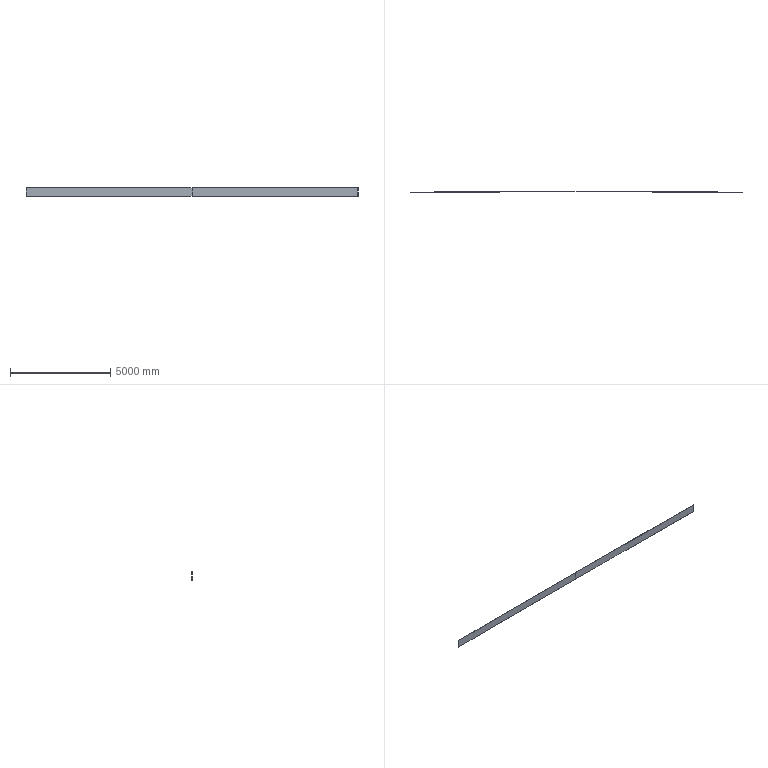Component | SolidWorks | UpperCover-1 | 1 solid | 8 faces | box 16590 x 30 x 400 mm | volume 66360064 mm3 | cylinder 4 | plane 4 | commonest cylinder face diameters 3440371.25 x2 3440351.25 x2 | material Plain Carbon Steel
STEP:
#1=COLOUR_RGB('',0.7922,0.8196,0.9333);
#2=FILL_AREA_STYLE_COLOUR('',#1);
#3=FILL_AREA_STYLE('',(#2));
#4=SURFACE_STYLE_FILL_AREA(#3);
#5=SURFACE_SIDE_STYLE('',(#4));
#6=SURFACE_STYLE_USAGE(.BOTH.,#5);
#7=PRESENTATION_STYLE_ASSIGNMENT((#6));
#8=CARTESIAN_POINT('',(18.305,126.764,80.917));
#9=VERTEX_POINT('',#8);
#10=CARTESIAN_POINT('',(344.879,127.551,80.917));
#11=VERTEX_POINT('',#10);
#12=CARTESIAN_POINT('',(344.879,-67596.292,80.917));
#13=DIRECTION('',(-0.,0.,-1.));
#14=DIRECTION('',(-0.,1.,0.));
#15=AXIS2_PLACEMENT_3D('',#12,#13,#14);
#16=CIRCLE('',#15,67723.844);
#17=EDGE_CURVE('',#9,#11,#16,.T.);
#18=ORIENTED_EDGE('',*,*,#17,.T.);
#19=CARTESIAN_POINT('',(344.879,127.551,65.169));
#20=VERTEX_POINT('',#19);
#21=CARTESIAN_POINT('',(344.879,127.551,80.917));
#22=DIRECTION('',(-0.,0.,-1.));
#23=VECTOR('',#22,39.37);
#24=LINE('',#21,#23);
#25=EDGE_CURVE('',#11,#20,#24,.T.);
#26=ORIENTED_EDGE('',*,*,#25,.T.);
#27=CARTESIAN_POINT('',(18.305,126.764,65.169));
#28=VERTEX_POINT('',#27);
#29=CARTESIAN_POINT('',(344.879,-67596.292,65.169));
#30=DIRECTION('',(-0.,0.,-1.));
#31=DIRECTION('',(-0.,1.,0.));
#32=AXIS2_PLACEMENT_3D('',#29,#30,#31);
#33=CIRCLE('',#32,67723.844);
#34=EDGE_CURVE('',#28,#20,#33,.T.);
#35=ORIENTED_EDGE('',*,*,#34,.F.);
#36=CARTESIAN_POINT('',(18.305,126.764,80.917));
#37=DIRECTION('',(-0.,0.,-1.));
#38=VECTOR('',#37,39.37);
#39=LINE('',#36,#38);
#40=EDGE_CURVE('',#9,#28,#39,.T.);
#41=ORIENTED_EDGE('',*,*,#40,.F.);
#42=EDGE_LOOP('',(#18,#26,#35,#41));
#43=FACE_OUTER_BOUND('',#42,.T.);
#44=CARTESIAN_POINT('',(344.879,-67596.292,80.917));
#45=DIRECTION('',(-0.,0.,-1.));
#46=DIRECTION('',(-0.,1.,0.));
#47=AXIS2_PLACEMENT_3D('',#44,#45,#46);
#48=CYLINDRICAL_SURFACE('',#47,67723.844);
#49=ADVANCED_FACE('',(#43),#48,.T.);
#50=CARTESIAN_POINT('',(344.879,127.158,80.917));
#51=VERTEX_POINT('',#50);
#52=CARTESIAN_POINT('',(671.452,126.37,80.917));
#53=VERTEX_POINT('',#52);
#54=CARTESIAN_POINT('',(344.879,-67596.292,80.917));
#55=DIRECTION('',(-0.,0.,-1.));
#56=DIRECTION('',(1.,0.,-0.));
#57=AXIS2_PLACEMENT_3D('',#54,#55,#56);
#58=CIRCLE('',#57,67723.45);
#59=EDGE_CURVE('',#51,#53,#58,.T.);
#60=ORIENTED_EDGE('',*,*,#59,.F.);
#61=CARTESIAN_POINT('',(344.879,127.158,65.169));
#62=VERTEX_POINT('',#61);
#63=CARTESIAN_POINT('',(344.879,127.158,80.917));
#64=DIRECTION('',(-0.,0.,-1.));
#65=VECTOR('',#64,39.37);
#66=LINE('',#63,#65);
#67=EDGE_CURVE('',#51,#62,#66,.T.);
#68=ORIENTED_EDGE('',*,*,#67,.T.);
#69=CARTESIAN_POINT('',(671.452,126.37,65.169));
#70=VERTEX_POINT('',#69);
#71=CARTESIAN_POINT('',(344.879,-67596.292,65.169));
#72=DIRECTION('',(-0.,0.,-1.));
#73=DIRECTION('',(1.,0.,-0.));
#74=AXIS2_PLACEMENT_3D('',#71,#72,#73);
#75=CIRCLE('',#74,67723.45);
#76=EDGE_CURVE('',#62,#70,#75,.T.);
#77=ORIENTED_EDGE('',*,*,#76,.T.);
#78=CARTESIAN_POINT('',(671.452,126.37,80.917));
#79=DIRECTION('',(-0.,0.,-1.));
#80=VECTOR('',#79,39.37);
#81=LINE('',#78,#80);
#82=EDGE_CURVE('',#53,#70,#81,.T.);
#83=ORIENTED_EDGE('',*,*,#82,.F.);
#84=EDGE_LOOP('',(#60,#68,#77,#83));
#85=FACE_OUTER_BOUND('',#84,.T.);
#86=CARTESIAN_POINT('',(344.879,-67596.292,80.917));
#87=DIRECTION('',(-0.,0.,-1.));
#88=DIRECTION('',(-0.,1.,0.));
#89=AXIS2_PLACEMENT_3D('',#86,#87,#88);
#90=CYLINDRICAL_SURFACE('',#89,67723.45);
#91=ADVANCED_FACE('',(#85),#90,.F.);
#92=ORIENTED_EDGE('',*,*,#67,.F.);
#93=CARTESIAN_POINT('',(18.307,126.37,80.917));
#94=VERTEX_POINT('',#93);
#95=CARTESIAN_POINT('',(344.879,-67596.292,80.917));
#96=DIRECTION('',(-0.,0.,-1.));
#97=DIRECTION('',(1.,0.,-0.));
#98=AXIS2_PLACEMENT_3D('',#95,#96,#97);
#99=CIRCLE('',#98,67723.45);
#100=EDGE_CURVE('',#94,#51,#99,.T.);
#101=ORIENTED_EDGE('',*,*,#100,.F.);
#102=CARTESIAN_POINT('',(18.307,126.37,65.169));
#103=VERTEX_POINT('',#102);
#104=CARTESIAN_POINT('',(18.307,126.37,80.917));
#105=DIRECTION('',(-0.,0.,-1.));
#106=VECTOR('',#105,39.37);
#107=LINE('',#104,#106);
#108=EDGE_CURVE('',#94,#103,#107,.T.);
#109=ORIENTED_EDGE('',*,*,#108,.T.);
#110=CARTESIAN_POINT('',(344.879,-67596.292,65.169));
#111=DIRECTION('',(-0.,0.,-1.));
#112=DIRECTION('',(1.,0.,-0.));
#113=AXIS2_PLACEMENT_3D('',#110,#111,#112);
#114=CIRCLE('',#113,67723.45);
#115=EDGE_CURVE('',#103,#62,#114,.T.);
#116=ORIENTED_EDGE('',*,*,#115,.T.);
#117=EDGE_LOOP('',(#92,#101,#109,#116));
#118=FACE_OUTER_BOUND('',#117,.T.);
#119=CARTESIAN_POINT('',(344.879,-67596.292,80.917));
#120=DIRECTION('',(-0.,0.,-1.));
#121=DIRECTION('',(-0.,1.,0.));
#122=AXIS2_PLACEMENT_3D('',#119,#120,#121);
#123=CYLINDRICAL_SURFACE('',#122,67723.45);
#124=ADVANCED_FACE('',(#118),#123,.F.);
#125=CARTESIAN_POINT('',(671.454,126.764,65.169));
#126=VERTEX_POINT('',#125);
#127=CARTESIAN_POINT('',(671.454,126.764,65.169));
#128=DIRECTION('',(-0.004822,-1.,-0.));
#129=VECTOR('',#128,39.37);
#130=LINE('',#127,#129);
#131=EDGE_CURVE('',#126,#70,#130,.T.);
#132=ORIENTED_EDGE('',*,*,#131,.F.);
#133=CARTESIAN_POINT('',(671.454,126.764,80.917));
#134=VERTEX_POINT('',#133);
#135=CARTESIAN_POINT('',(671.454,126.764,80.917));
#136=DIRECTION('',(-0.,0.,-1.));
#137=VECTOR('',#136,39.37);
#138=LINE('',#135,#137);
#139=EDGE_CURVE('',#134,#126,#138,.T.);
#140=ORIENTED_EDGE('',*,*,#139,.F.);
#141=CARTESIAN_POINT('',(671.454,126.764,80.917));
#142=DIRECTION('',(-0.004822,-1.,-0.));
#143=VECTOR('',#142,39.37);
#144=LINE('',#141,#143);
#145=EDGE_CURVE('',#134,#53,#144,.T.);
#146=ORIENTED_EDGE('',*,*,#145,.T.);
#147=ORIENTED_EDGE('',*,*,#82,.T.);
#148=EDGE_LOOP('',(#132,#140,#146,#147));
#149=FACE_OUTER_BOUND('',#148,.T.);
#150=CARTESIAN_POINT('',(671.454,126.764,80.917));
#151=DIRECTION('',(1.,-0.004822,-0.));
#152=DIRECTION('',(0.004822,1.,0.));
#153=AXIS2_PLACEMENT_3D('',#150,#151,#152);
#154=PLANE('',#153);
#155=ADVANCED_FACE('',(#149),#154,.T.);
#156=ORIENTED_EDGE('',*,*,#25,.F.);
#157=CARTESIAN_POINT('',(344.879,-67596.292,80.917));
#158=DIRECTION('',(-0.,0.,-1.));
#159=DIRECTION('',(-0.,1.,0.));
#160=AXIS2_PLACEMENT_3D('',#157,#158,#159);
#161=CIRCLE('',#160,67723.844);
#162=EDGE_CURVE('',#11,#134,#161,.T.);
#163=ORIENTED_EDGE('',*,*,#162,.T.);
#164=ORIENTED_EDGE('',*,*,#139,.T.);
#165=CARTESIAN_POINT('',(344.879,-67596.292,65.169));
#166=DIRECTION('',(-0.,0.,-1.));
#167=DIRECTION('',(-0.,1.,0.));
#168=AXIS2_PLACEMENT_3D('',#165,#166,#167);
#169=CIRCLE('',#168,67723.844);
#170=EDGE_CURVE('',#20,#126,#169,.T.);
#171=ORIENTED_EDGE('',*,*,#170,.F.);
#172=EDGE_LOOP('',(#156,#163,#164,#171));
#173=FACE_OUTER_BOUND('',#172,.T.);
#174=CARTESIAN_POINT('',(344.879,-67596.292,80.917));
#175=DIRECTION('',(-0.,0.,-1.));
#176=DIRECTION('',(-0.,1.,0.));
#177=AXIS2_PLACEMENT_3D('',#174,#175,#176);
#178=CYLINDRICAL_SURFACE('',#177,67723.844);
#179=ADVANCED_FACE('',(#173),#178,.T.);
#180=CARTESIAN_POINT('',(18.307,126.37,65.169));
#181=DIRECTION('',(-0.004822,1.,0.));
#182=VECTOR('',#181,39.37);
#183=LINE('',#180,#182);
#184=EDGE_CURVE('',#103,#28,#183,.T.);
#185=ORIENTED_EDGE('',*,*,#184,.F.);
#186=ORIENTED_EDGE('',*,*,#108,.F.);
#187=CARTESIAN_POINT('',(18.307,126.37,80.917));
#188=DIRECTION('',(-0.004822,1.,0.));
#189=VECTOR('',#188,39.37);
#190=LINE('',#187,#189);
#191=EDGE_CURVE('',#94,#9,#190,.T.);
#192=ORIENTED_EDGE('',*,*,#191,.T.);
#193=ORIENTED_EDGE('',*,*,#40,.T.);
#194=EDGE_LOOP('',(#185,#186,#192,#193));
#195=FACE_OUTER_BOUND('',#194,.T.);
#196=CARTESIAN_POINT('',(18.307,126.37,80.917));
#197=DIRECTION('',(-1.,-0.004822,0.));
#198=DIRECTION('',(0.004822,-1.,-0.));
#199=AXIS2_PLACEMENT_3D('',#196,#197,#198);
#200=PLANE('',#199);
#201=ADVANCED_FACE('',(#195),#200,.T.);
#202=ORIENTED_EDGE('',*,*,#100,.T.);
#203=ORIENTED_EDGE('',*,*,#59,.T.);
#204=ORIENTED_EDGE('',*,*,#145,.F.);
#205=ORIENTED_EDGE('',*,*,#162,.F.);
#206=ORIENTED_EDGE('',*,*,#17,.F.);
#207=ORIENTED_EDGE('',*,*,#191,.F.);
#208=EDGE_LOOP('',(#202,#203,#204,#205,#206,#207));
#209=FACE_OUTER_BOUND('',#208,.T.);
#210=CARTESIAN_POINT('',(344.879,-67596.292,80.917));
#211=DIRECTION('',(0.,-0.,1.));
#212=DIRECTION('',(1.,0.,-0.));
#213=AXIS2_PLACEMENT_3D('',#210,#211,#212);
#214=PLANE('',#213);
#215=ADVANCED_FACE('',(#209),#214,.T.);
#216=ORIENTED_EDGE('',*,*,#115,.F.);
#217=ORIENTED_EDGE('',*,*,#184,.T.);
#218=ORIENTED_EDGE('',*,*,#34,.T.);
#219=ORIENTED_EDGE('',*,*,#170,.T.);
#220=ORIENTED_EDGE('',*,*,#131,.T.);
#221=ORIENTED_EDGE('',*,*,#76,.F.);
#222=EDGE_LOOP('',(#216,#217,#218,#219,#220,#221));
#223=FACE_OUTER_BOUND('',#222,.T.);
#224=CARTESIAN_POINT('',(344.879,-67596.292,65.169));
#225=DIRECTION('',(0.,-0.,1.));
#226=DIRECTION('',(1.,0.,-0.));
#227=AXIS2_PLACEMENT_3D('',#224,#225,#226);
#228=PLANE('',#227);
#229=ADVANCED_FACE('',(#223),#228,.F.);
#230=CLOSED_SHELL('',(#49,#91,#124,#155,#179,#201,#215,#229));
#231=MANIFOLD_SOLID_BREP('',#230);
#232=STYLED_ITEM('',(#7),#231);
#233=(LENGTH_UNIT()NAMED_UNIT(*)SI_UNIT($,.METRE.));
#234=LENGTH_MEASURE_WITH_UNIT(LENGTH_MEASURE(0.0254),#233);
#235=DIMENSIONAL_EXPONENTS(1.,0.,0.,0.,0.,0.,0.);
#236=(CONVERSION_BASED_UNIT('',#234)LENGTH_UNIT()NAMED_UNIT(#235));
#237=UNCERTAINTY_MEASURE_WITH_UNIT(LENGTH_MEASURE(0.00001),#236,'','');
#238=(NAMED_UNIT(*)PLANE_ANGLE_UNIT()SI_UNIT($,.RADIAN.));
#239=(NAMED_UNIT(*)SI_UNIT($,.STERADIAN.)SOLID_ANGLE_UNIT());
#240=(GEOMETRIC_REPRESENTATION_CONTEXT(3)GLOBAL_UNCERTAINTY_ASSIGNED_CONTEXT((#237))GLOBAL_UNIT_ASSIGNED_CONTEXT((#236,#238,#239))REPRESENTATION_CONTEXT('',''));
#241=MECHANICAL_DESIGN_GEOMETRIC_PRESENTATION_REPRESENTATION('',(#232),#240);
#242=CARTESIAN_POINT('',(0.,0.,0.));
#243=DIRECTION('',(0.,0.,1.));
#244=DIRECTION('',(1.,0.,0.));
#245=AXIS2_PLACEMENT_3D('',#242,#243,#244);
#246=(LENGTH_UNIT()NAMED_UNIT(*)SI_UNIT($,.METRE.));
#247=LENGTH_MEASURE_WITH_UNIT(LENGTH_MEASURE(0.0254),#246);
#248=DIMENSIONAL_EXPONENTS(1.,0.,0.,0.,0.,0.,0.);
#249=(CONVERSION_BASED_UNIT('',#247)LENGTH_UNIT()NAMED_UNIT(#248));
#250=UNCERTAINTY_MEASURE_WITH_UNIT(LENGTH_MEASURE(0.00001),#249,'','');
#251=(NAMED_UNIT(*)PLANE_ANGLE_UNIT()SI_UNIT($,.RADIAN.));
#252=(NAMED_UNIT(*)SI_UNIT($,.STERADIAN.)SOLID_ANGLE_UNIT());
#253=(GEOMETRIC_REPRESENTATION_CONTEXT(3)GLOBAL_UNCERTAINTY_ASSIGNED_CONTEXT((#250))GLOBAL_UNIT_ASSIGNED_CONTEXT((#249,#251,#252))REPRESENTATION_CONTEXT('',''));
#254=ADVANCED_BREP_SHAPE_REPRESENTATION('',(#231,#245),#253);
#255=PRESENTATION_LAYER_ASSIGNMENT('','',(#232));